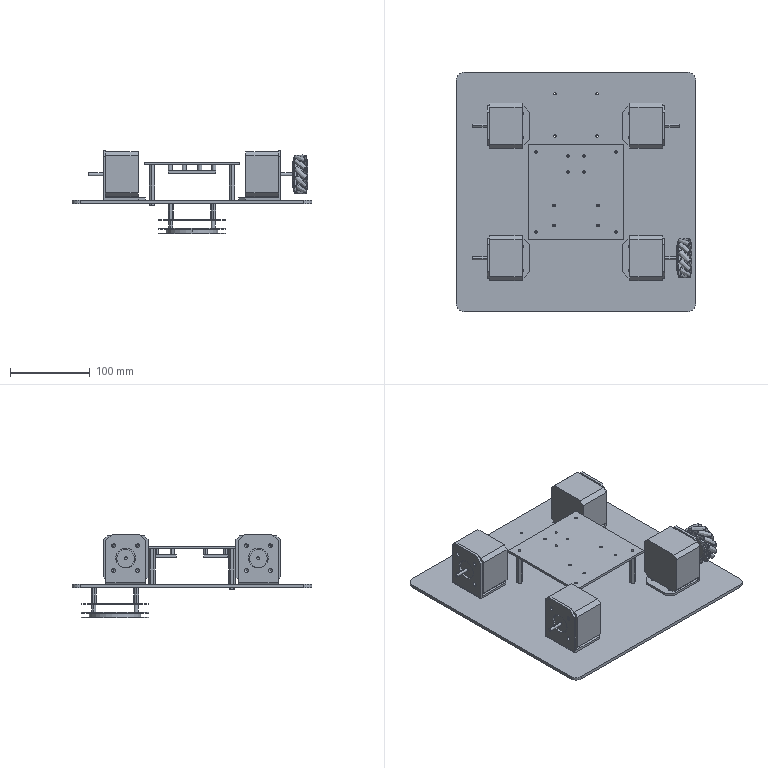Assembly | SolidWorks | mm | 38 component files | 41 solids | 1139 faces | box 300 x 300 x 105 mm | volume 1042344 mm3 | cylinder 602 | plane 303 | cone 204 | spline 24 | torus 6 | commonest cylinder face diameters 3 x182 5 x88 4 x72 3.2 x60 4.2 x56 16 x34 1.6 x24 2 x24
Bill of materials:
25CopperPillar-Copy | 4 |  | Long slender hexagonal prism with a single round axial bore running through it; looks like a hex standoff/spacer.
42StepperMotor | 4 |  | Roughly cubic rectangular body with chamfered vertical edges, a short round boss on one face and a small cylindrical shaft sticking out from the boss.
10CopperPillar | 8 |  | Plain cylindrical tube/sleeve with a concentric through bore and flat ends; length is greater than outer diameter.
Plate2 | 1 |  | Square flat plate of moderate thickness with four round through-holes, one near each corner.
Plate2555 | 1 |  | Rectangular flat plate, about 2:1 aspect ratio, with four small round through-holes near the corners.
Plate3 | 1 |  | Thin square plate with sharp corners and 12 small round through-holes: one at each corner, a small square group of four in the upper middle, and a wider rectangular group of four in the lower middle.
Chassis | 1 |  | Thin square plate with rounded corners, carrying several groups of small through-holes: four 2x2 square hole groups near the corners plus smaller holes arranged symmetrically between them.
GB_T5781-2000HexHeadBoltFullThreadGradeCM5_30 | 1 |  | Hex-head bolt/screw with an integral washer face or flange under the head, a fully threaded cylindrical shank and a chamfered tip.
10Pillar | 4 |  | Plain cylindrical tube/sleeve with a concentric through bore and flat ends; proportions differ slightly from the similar sleeve (relatively thicker wall).
20Pillars | 4 |  | Hexagonal prism with a large round axial bore; shorter and with a relatively larger bore than the long hex part, like a hex standoff or coupling.
Gimbal1 | 3 |  | Thin circular disc with a narrow concentric annular gap separating an outer ring from an inner disc. The outer ring has four holes. The inner disc has four holes on a circle plus a central hole surrounded by four smaller holes.
GimbalMiddle | 1 |  | Flat circular disc of moderate thickness with four equally spaced round through-holes on a bolt-circle-like pattern near the rim.
MecanumWheel | 1 |  | Wheel-like body that is round when seen along its axis. It has a central hub disc with a large plain round through-bore. Around the edge sits a ring of evenly spaced, barrel-shaped rollers set at an angle to the axis, held by curved, hook-shaped side supports. The overall layout looks like a mecanum-style wheel.
Mount | 4 |  | L-shaped bracket made from thin plate of constant thickness, with a 90-degree bend and a small inside corner radius. The upright flange has a large central round hole with four smaller round holes in a rectangular pattern around it, and its two outer corners are cut at an angle. The base flange has two long parallel slots with rounded ends and two angled corner cuts at its free edge. The layout fits a face-mount bracket with slots for adjusting position.
Mates:
1. coincident | Chassis-1 face at (140, -140, 4) dir (0, 0, 1) | Mount-1 face at (-111.419, 83, 4) dir (0, 0, -1)
2. concentric | Chassis-1 face at (-98, 98, 4) dir (0, 0, -1) r 2.1 | Mount-1 face at (-98, 98, 4) dir (0, 0, 1) r 2.1
3. concentric | Chassis-1 face at (-98, 68, 4) dir (0, 0, -1) r 2.1 | Mount-1 face at (-98, 68, 4) dir (0, 0, 1) r 2.1
4. concentric | Mount-1 face at (-108.419, 98, 21.5) dir (-1, 0, 0) r 2.5 | 42StepperMotor-2 face at (-108.419, 98, 21.5) dir (-1, 0, 0) r 2.5
5. concentric | Mount-1 face at (-108.419, 68, 21.5) dir (-1, 0, 0) r 2.5 | 42StepperMotor-2 face at (-108.419, 68, 21.5) dir (-1, 0, 0) r 2.5
6. coincident | Chassis-1 face at (140, -140, 4) dir (0, 0, 1) | Mount-7 face at (111.398, -83, 4) dir (0, 0, -1)
7. concentric | Chassis-1 face at (68, -68, 4) dir (0, 0, -1) r 2.1 | Mount-7 face at (68, -68, 4) dir (0, 0, 1) r 2.1
8. concentric | Chassis-1 face at (68, -98, 4) dir (0, 0, -1) r 2.1 | Mount-7 face at (68, -98, 4) dir (0, 0, 1) r 2.1
9. coincident | Mount-7 face at (108.398, -83, 37) dir (-1, 0, 0) | 42StepperMotor-5 face at (108.398, -83, 36.5) dir (1, 0, 0)
10. concentric | Mount-7 face at (108.398, -68, 21.5) dir (1, 0, 0) r 2.5 | 42StepperMotor-5 face at (108.398, -68, 21.5) dir (1, 0, 0) r 2.5
11. concentric | Mount-7 face at (108.398, -98, 21.5) dir (1, 0, 0) r 2.5 | 42StepperMotor-5 face at (108.398, -98, 21.5) dir (1, 0, 0) r 2.5
12. coincident | Mount-1 face at (-108.419, 83, 37) dir (1, 0, 0) | 42StepperMotor-2 face at (-108.419, 83, 36.5) dir (-1, 0, 0)
13. concentric | Chassis-1 face at (50, 50, -6) dir (0, 0, 1) r 1.5 | 25CopperPillar-Copy-1 face at (50, 50, 49) dir (0, 0, -1) r 1.6
14. concentric | 25CopperPillar-Copy-2 face at (-50, 50, 49) dir (0, 0, -1) r 1.6 | Assembly3-1/Plate3-1 face at (-50, 50, 52) dir (0, 0, -1) r 1.5
15. concentric | 25CopperPillar-Copy-1 face at (50, 50, 49) dir (0, 0, -1) r 1.6 | Assembly3-1/Plate3-1 face at (50, 50, 52) dir (0, 0, -1) r 1.5
16. coincident | Chassis-1 face at (140, -140, 4) dir (0, 0, 1) | 25CopperPillar-Copy-1 face at (50, 50, 4) dir (0, 0, -1)
17. coincident | 25CopperPillar-Copy-1 face at (50, 50, 49) dir (0, 0, 1) | Assembly3-1/Plate3-1 face at (0, 0, 49) dir (0, 0, -1)
18. coincident | Chassis-1 face at (140, -140, 0) dir (0, 0, -1) | GB_T5781-2000HexHeadBoltFullThreadGradeCM5_30-1 face at (-49.888, -46.827, 0) dir (0, 0, 1)
19. concentric | Chassis-1 face at (-50, -50, -6) dir (0, 0, 1) r 1.5 | GB_T5781-2000HexHeadBoltFullThreadGradeCM5_30-1 face at (-50, -50, -2) dir (0, 0, -1) r 2.75
20. concentric | 42StepperMotor-5 face at (129.398, -83, 36.5) dir (-1, 0, 0) r 1.875 | MecanumWheel-1 face at (135.798, -83, 36.5) dir (-1, 0, 0) r 8
21. distance | Mount-7 face at (111.398, -83, 37) dir (1, 0, 0) | MecanumWheel-1 face at (126.398, -90.961, 37.29) dir (-1, 0, 0)
22. coincident | Chassis-1 face at (140, -140, 0) dir (0, 0, -1) | Gimbal-1/20Pillars-3 face at (-26.5, 123, 0) dir (0, 0, 1)
23. concentric | Chassis-1 face at (-26.5, 70, -16) dir (0, 0, 1) r 1.5 | Gimbal-1/20Pillars-2 face at (-26.5, 70, -20) dir (0, 0, 1) r 1.5
24. concentric | Chassis-1 face at (-26.5, 123, -16) dir (0, 0, 1) r 1.5 | Gimbal-1/10Pillar-2 face at (-26.5, 123, -31) dir (0, 0, 1) r 2.5
25. concentric | Plate3-1 face at (-10, -45, -7) dir (0, 0, 1) r 1.5 | 10CopperPillar-1 face at (-10, -45, 11) dir (0, 0, -1) r 1.6
26. coincident | Plate3-1 face at (0, 0, 3) dir (0, 0, 1) | 10CopperPillar-1 face at (-10, -45, 3) dir (0, 0, -1)
27. concentric | Plate3-1 face at (-27.5, 42, -7) dir (0, 0, 1) r 1.5 | 10CopperPillar-9 face at (-27.5, 42, 11) dir (0, 0, -1) r 1.6
28. coincident | Plate3-1 face at (0, 0, 3) dir (0, 0, 1) | 10CopperPillar-9 face at (-27.5, 42, 3) dir (0, 0, -1)
29. coincident | Plate2555-1 face at (0, 29.5, 11) dir (0, 0, -1) | 10CopperPillar-10 face at (-27.5, 17, 11) dir (0, 0, 1)
30. concentric | Plate2555-1 face at (-27.5, 17, 14) dir (0, 0, -1) r 1.118 | 10CopperPillar-10 face at (-27.5, 17, 11) dir (0, 0, -1) r 1.6
31. concentric | Plate2555-1 face at (-27.5, 42, 14) dir (0, 0, -1) r 1.118 | 10CopperPillar-9 face at (-27.5, 42, 11) dir (0, 0, -1) r 1.6
32. coincident | 10CopperPillar-1 face at (-10, -45, 11) dir (0, 0, 1) | Plate2-1 face at (0, -35, 11) dir (0, 0, -1)
33. concentric | 10CopperPillar-1 face at (-10, -45, 11) dir (0, 0, -1) r 1.6 | Plate2-1 face at (-10, -45, 14) dir (0, 0, -1) r 1.5
34. concentric | Plate2-1 face at (-10, -25, 14) dir (0, 0, -1) r 1.5 | 10CopperPillar-6 face at (-10, -25, 11) dir (0, 0, -1) r 1.6
35. coincident | Gimbal1-1 face at (-4.24, 1.749, 0) dir (0, 0, -1) | GimbalMiddle-1 face at (-4.24, 1.749, 0) dir (0, 0, 1)
36. concentric | Gimbal1-1 face at (-4.24, -23.251, -9) dir (0, 0, 1) r 1.5 | GimbalMiddle-1 face at (-4.24, -23.251, -10) dir (0, 0, 1) r 1.5
37. concentric | Gimbal1-1 face at (20.76, 1.749, -9) dir (0, 0, 1) r 1.5 | GimbalMiddle-1 face at (20.76, 1.749, -10) dir (0, 0, 1) r 1.5
38. coincident | GimbalMiddle-1 face at (-4.24, 1.749, -5) dir (0, 0, -1) | Gimbal1-2 face at (-4.24, 1.749, -5) dir (0, 0, 1)
39. concentric | GimbalMiddle-1 face at (-29.24, 1.749, -10) dir (0, 0, 1) r 1.5 | Gimbal1-2 edge at (-29.24, 1.749, -6) dir (0, 0, 1) r 1.5
40. concentric | GimbalMiddle-1 face at (-4.24, -23.251, -10) dir (0, 0, 1) r 1.5 | Gimbal1-2 face at (-4.24, -23.251, -15) dir (0, 0, 1) r 1.5
41. concentric | GimbalMiddle-1 face at (20.76, 1.749, -10) dir (0, 0, 1) r 1.5 | Gimbal1-2 face at (20.76, 1.749, -15) dir (0, 0, 1) r 1.5
42. coincident | Gimbal1-2 face at (-4.24, 1.749, -6) dir (0, 0, -1) | 10Pillar-1 face at (22.26, 28.249, -6) dir (0, 0, 1)
43. concentric | Gimbal1-2 face at (22.26, 28.249, -6) dir (0, 0, 1) r 1.5 | 10Pillar-1 face at (22.26, 28.249, -6) dir (0, 0, -1) r 1.5
44. coincident | 10Pillar-4 face at (22.26, -24.751, -16) dir (0, 0, -1) | Gimbal1-3 face at (-4.24, 1.749, -16) dir (0, 0, 1)
45. concentric | 10Pillar-4 face at (22.26, -24.751, -6) dir (0, 0, -1) r 1.5 | Gimbal1-3 face at (22.26, -24.751, -17) dir (0, 0, 1) r 1.5
46. concentric | 10Pillar-3 face at (-30.74, -24.751, -6) dir (0, 0, -1) r 1.5 | Gimbal1-3 face at (-30.74, -24.751, -17) dir (0, 0, 1) r 1.5
47. coincident | Gimbal1-3 face at (-4.24, 1.749, -17) dir (0, 0, -1) | 20Pillars-1 face at (22.26, -24.751, -17) dir (0, 0, 1)
48. concentric | Gimbal1-3 face at (22.26, -24.751, -17) dir (0, 0, 1) r 1.5 | 20Pillars-1 face at (22.26, -24.751, -17) dir (0, 0, -1) r 1.5